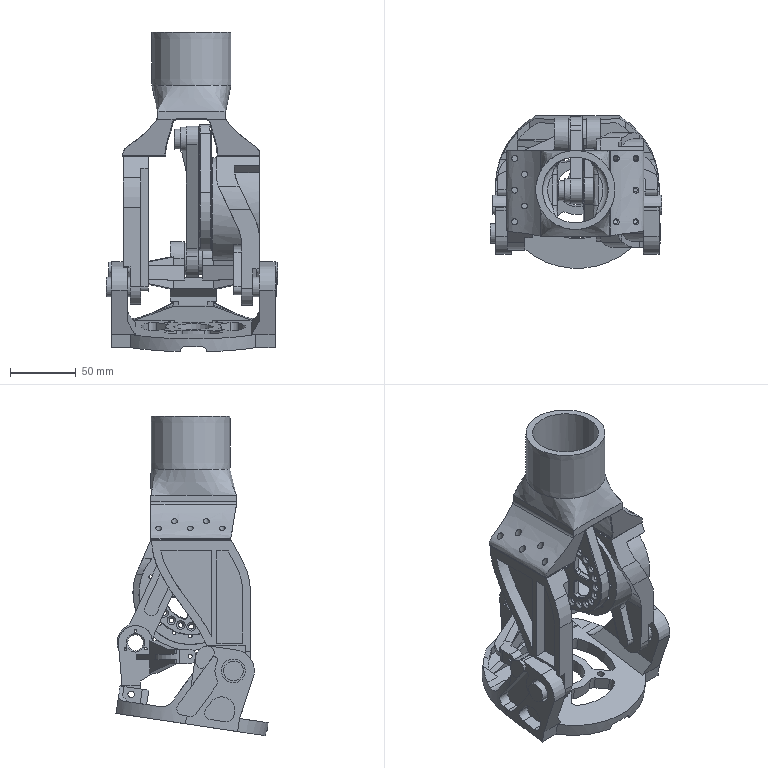Assembly | NX | mm | 7 component files | 7 solids | 639 faces | box 130 x 115.45 x 242.12 mm | volume 475130 mm3 | cylinder 262 | plane 258 | torus 65 | cone 22 | spline 19 | other 8 | sphere 5 | commonest cylinder face diameters 1 x39 8 x24 3.5 x20 4 x16 2.7 x16 10 x13 12 x10 4.5 x10
Bill of materials:
unnamed part 1 | 1 |  | Symmetric forked bracket. Two coaxial cylindrical bosses with bores sit side by side with a gap between them. From them, two tapered arms run out to the sides and end in flat tabs with small holes.
unnamed part 2 | 1 |  | Saddle-style base with a vertical tube on top. The thin-walled tube rises from a body that flares out into two angled, curved mounting flanges, each drilled with a hole pattern. The underside has an opening with straight sides.
unnamed part 3 | 1 |  | Straight link: a flat bar with a ring-shaped boss at each end. The two bosses are offset from each other across the bar's thickness.
unnamed part 4 | 1 |  | Mostly round mounting plate with a large central bore and four curved lightening cutouts. A small hole sits between each pair of cutouts. Two upright side brackets, each with a large through-hole, stand on opposite sides, and a ribbed hollow-box reinforcement runs along one edge.
unnamed part 5 | 1 |  | Ring housing with a lever arm. A wide cylindrical ring has a large bore and a circle of small holes on its face. A flat rectangular pad with a small hole pattern sits on top. A curved arm extends down from the ring and ends in a short cylindrical pin.
unnamed part 6 | 1 |  | Curved, tapering plate shaped like a tooth or paddle. One edge carries a stepped flange, and a short cylindrical pin sticks out near the rounded lower end.
unnamed part 7 | 1 |  | Teardrop-shaped plate with a raised rim. A circle of small holes and four quadrant-shaped cutouts separated by a cross of spokes sit in the round end. A cylindrical pin sticks out from the back face near the round end.
Mates:
1. touch align | Tilt_Base_Acc_2 1 face | Tilt_RotorRod_Conn_Mnt 1 face
2. touch align | Tilt_Base_Acc_2 1 edge | Tilt_RotorRod_Conn_Mnt 1 edge
3. touch align | Tilt_Base_Acc_2 1 edge | Tilt_RotorRod_Conn_Mnt 1 edge
4. touch align | Link_Rod 1 face | Motor_Drive_Rod 1 face
5. touch align | Link_Rod 1 face | Motor_Drive_Rod 1 face
6. fix | Motor_Drive_Rod 1 component
7. fix | Tilt_RotorRod_Conn_Mnt 1 component
8. touch align | Tilt_Base_Acc_1 1 face | Tilt_RotorRod_Conn_Mnt 1 face
9. touch align | Tilt_Base_Acc_1 1 edge | Tilt_RotorRod_Conn_Mnt 1 edge
10. touch align | Tilt_Base_Acc_1 1 edge | Tilt_RotorRod_Conn_Mnt 1 edge
11. touch align | Rotor_Base_Acc 1 face | Rotor_Base 1 face
12. touch align | Rotor_Base_Acc 1 face | Rotor_Base 1 face
13. touch align | Rotor_Base 1 face | Tilt_Base_Acc_2 1 face
14. distance | Tilt_Base_Acc_2 1 face | Rotor_Base 1 edge
15. touch align | Link_Rod 1 face | Rotor_Base_Acc 1 face